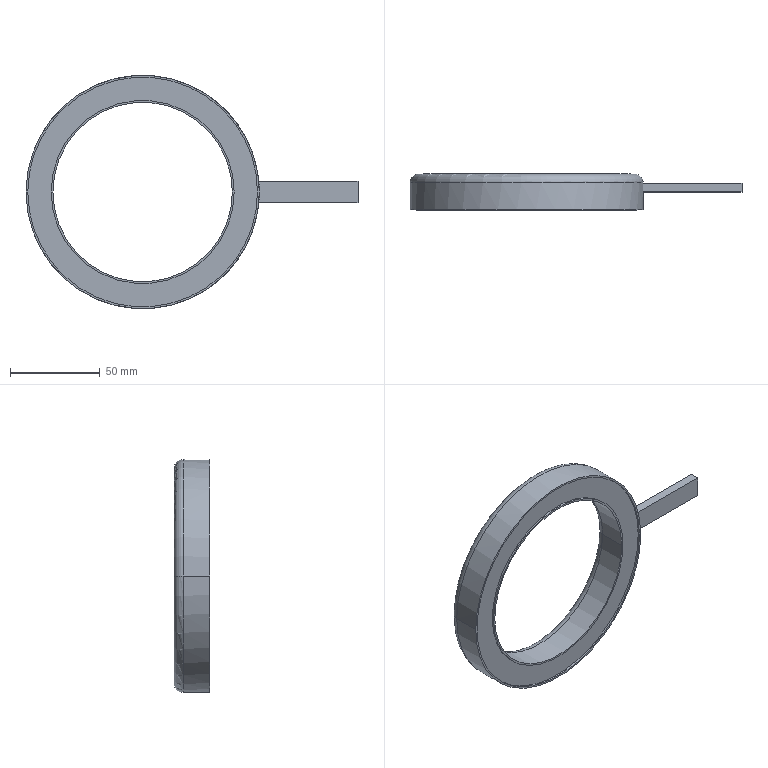Component | SolidWorks | FillLight-1 | 1 solid | 21 faces | box 185 x 20 x 130 mm | volume 103117 mm3 | plane 9 | cylinder 8 | torus 4 | commonest cylinder face diameters 102 x2 128 x2 100 x2 130 x2
STEP:
#1=CARTESIAN_POINT('',(8.917,22.343,-0.));
#2=VERTEX_POINT('',#1);
#3=CARTESIAN_POINT('',(4.902,22.343,-0.));
#4=VERTEX_POINT('',#3);
#5=CARTESIAN_POINT('',(6.909,22.343,-0.));
#6=DIRECTION('',(-0.,-1.,0.));
#7=DIRECTION('',(1.,0.,0.));
#8=AXIS2_PLACEMENT_3D('',#5,#6,#7);
#9=CIRCLE('',#8,2.008);
#10=EDGE_CURVE('',#2,#4,#9,.T.);
#11=ORIENTED_EDGE('',*,*,#10,.T.);
#12=CARTESIAN_POINT('',(4.902,22.303,-0.));
#13=VERTEX_POINT('',#12);
#14=CARTESIAN_POINT('',(4.902,22.343,-0.));
#15=DIRECTION('',(-0.,-1.,0.));
#16=VECTOR('',#15,39.37);
#17=LINE('',#14,#16);
#18=EDGE_CURVE('',#4,#13,#17,.T.);
#19=ORIENTED_EDGE('',*,*,#18,.T.);
#20=CARTESIAN_POINT('',(8.917,22.303,-0.));
#21=VERTEX_POINT('',#20);
#22=CARTESIAN_POINT('',(6.909,22.303,-0.));
#23=DIRECTION('',(-0.,-1.,0.));
#24=DIRECTION('',(1.,0.,0.));
#25=AXIS2_PLACEMENT_3D('',#22,#23,#24);
#26=CIRCLE('',#25,2.008);
#27=EDGE_CURVE('',#21,#13,#26,.T.);
#28=ORIENTED_EDGE('',*,*,#27,.F.);
#29=CARTESIAN_POINT('',(8.917,22.343,-0.));
#30=DIRECTION('',(-0.,-1.,0.));
#31=VECTOR('',#30,39.37);
#32=LINE('',#29,#31);
#33=EDGE_CURVE('',#2,#21,#32,.T.);
#34=ORIENTED_EDGE('',*,*,#33,.F.);
#35=EDGE_LOOP('',(#11,#19,#28,#34));
#36=FACE_OUTER_BOUND('',#35,.T.);
#37=CARTESIAN_POINT('',(6.909,22.343,-0.));
#38=DIRECTION('',(-0.,-1.,0.));
#39=DIRECTION('',(1.,0.,0.));
#40=AXIS2_PLACEMENT_3D('',#37,#38,#39);
#41=CYLINDRICAL_SURFACE('',#40,2.008);
#42=ADVANCED_FACE('',(#36),#41,.T.);
#43=CARTESIAN_POINT('',(4.39,22.343,-0.));
#44=VERTEX_POINT('',#43);
#45=CARTESIAN_POINT('',(9.429,22.343,-0.));
#46=VERTEX_POINT('',#45);
#47=CARTESIAN_POINT('',(6.909,22.343,-0.));
#48=DIRECTION('',(-0.,-1.,0.));
#49=DIRECTION('',(1.,0.,0.));
#50=AXIS2_PLACEMENT_3D('',#47,#48,#49);
#51=CIRCLE('',#50,2.52);
#52=EDGE_CURVE('',#44,#46,#51,.T.);
#53=ORIENTED_EDGE('',*,*,#52,.F.);
#54=CARTESIAN_POINT('',(4.39,22.303,-0.));
#55=VERTEX_POINT('',#54);
#56=CARTESIAN_POINT('',(4.39,22.343,-0.));
#57=DIRECTION('',(-0.,-1.,0.));
#58=VECTOR('',#57,39.37);
#59=LINE('',#56,#58);
#60=EDGE_CURVE('',#44,#55,#59,.T.);
#61=ORIENTED_EDGE('',*,*,#60,.T.);
#62=CARTESIAN_POINT('',(9.429,22.303,-0.));
#63=VERTEX_POINT('',#62);
#64=CARTESIAN_POINT('',(6.909,22.303,-0.));
#65=DIRECTION('',(-0.,-1.,0.));
#66=DIRECTION('',(1.,0.,0.));
#67=AXIS2_PLACEMENT_3D('',#64,#65,#66);
#68=CIRCLE('',#67,2.52);
#69=EDGE_CURVE('',#55,#63,#68,.T.);
#70=ORIENTED_EDGE('',*,*,#69,.T.);
#71=CARTESIAN_POINT('',(9.429,22.343,-0.));
#72=DIRECTION('',(-0.,-1.,0.));
#73=VECTOR('',#72,39.37);
#74=LINE('',#71,#73);
#75=EDGE_CURVE('',#46,#63,#74,.T.);
#76=ORIENTED_EDGE('',*,*,#75,.F.);
#77=EDGE_LOOP('',(#53,#61,#70,#76));
#78=FACE_OUTER_BOUND('',#77,.T.);
#79=CARTESIAN_POINT('',(6.909,22.343,-0.));
#80=DIRECTION('',(-0.,-1.,0.));
#81=DIRECTION('',(1.,0.,0.));
#82=AXIS2_PLACEMENT_3D('',#79,#80,#81);
#83=CYLINDRICAL_SURFACE('',#82,2.52);
#84=ADVANCED_FACE('',(#78),#83,.F.);
#85=CARTESIAN_POINT('',(9.075,23.091,-0.));
#86=VERTEX_POINT('',#85);
#87=CARTESIAN_POINT('',(4.744,23.091,-0.));
#88=VERTEX_POINT('',#87);
#89=CARTESIAN_POINT('',(6.909,23.091,-0.));
#90=DIRECTION('',(-0.,-1.,0.));
#91=DIRECTION('',(-1.,0.,0.));
#92=AXIS2_PLACEMENT_3D('',#89,#90,#91);
#93=CIRCLE('',#92,2.165);
#94=EDGE_CURVE('',#86,#88,#93,.T.);
#95=ORIENTED_EDGE('',*,*,#94,.F.);
#96=CARTESIAN_POINT('',(8.878,22.894,-0.));
#97=VERTEX_POINT('',#96);
#98=CARTESIAN_POINT('',(9.075,22.894,-0.));
#99=DIRECTION('',(-0.,0.,1.));
#100=DIRECTION('',(1.,0.,0.));
#101=AXIS2_PLACEMENT_3D('',#98,#99,#100);
#102=CIRCLE('',#101,0.1969);
#103=EDGE_CURVE('',#86,#97,#102,.T.);
#104=ORIENTED_EDGE('',*,*,#103,.T.);
#105=CARTESIAN_POINT('',(4.941,22.894,-0.));
#106=VERTEX_POINT('',#105);
#107=CARTESIAN_POINT('',(6.909,22.894,-0.));
#108=DIRECTION('',(0.,1.,0.));
#109=DIRECTION('',(-1.,0.,0.));
#110=AXIS2_PLACEMENT_3D('',#107,#108,#109);
#111=CIRCLE('',#110,1.969);
#112=EDGE_CURVE('',#106,#97,#111,.T.);
#113=ORIENTED_EDGE('',*,*,#112,.F.);
#114=CARTESIAN_POINT('',(4.744,22.894,-0.));
#115=DIRECTION('',(0.,-0.,-1.));
#116=DIRECTION('',(-1.,0.,0.));
#117=AXIS2_PLACEMENT_3D('',#114,#115,#116);
#118=CIRCLE('',#117,0.1969);
#119=EDGE_CURVE('',#88,#106,#118,.T.);
#120=ORIENTED_EDGE('',*,*,#119,.F.);
#121=EDGE_LOOP('',(#95,#104,#113,#120));
#122=FACE_OUTER_BOUND('',#121,.T.);
#123=CARTESIAN_POINT('',(6.909,22.894,-0.));
#124=DIRECTION('',(0.,1.,0.));
#125=DIRECTION('',(-1.,0.,0.));
#126=AXIS2_PLACEMENT_3D('',#123,#124,#125);
#127=TOROIDAL_SURFACE('',#126,2.165,0.1969);
#128=ADVANCED_FACE('',(#122),#127,.T.);
#129=CARTESIAN_POINT('',(9.458,22.894,0.2362));
#130=VERTEX_POINT('',#129);
#131=CARTESIAN_POINT('',(9.469,22.894,-0.));
#132=VERTEX_POINT('',#131);
#133=CARTESIAN_POINT('',(6.909,22.894,-0.));
#134=DIRECTION('',(0.,1.,0.));
#135=DIRECTION('',(-1.,0.,0.));
#136=AXIS2_PLACEMENT_3D('',#133,#134,#135);
#137=CIRCLE('',#136,2.559);
#138=EDGE_CURVE('',#130,#132,#137,.T.);
#139=ORIENTED_EDGE('',*,*,#138,.T.);
#140=CARTESIAN_POINT('',(9.272,23.091,-0.));
#141=VERTEX_POINT('',#140);
#142=CARTESIAN_POINT('',(9.272,22.894,-0.));
#143=DIRECTION('',(-0.,0.,1.));
#144=DIRECTION('',(1.,0.,0.));
#145=AXIS2_PLACEMENT_3D('',#142,#143,#144);
#146=CIRCLE('',#145,0.1969);
#147=EDGE_CURVE('',#132,#141,#146,.T.);
#148=ORIENTED_EDGE('',*,*,#147,.T.);
#149=CARTESIAN_POINT('',(4.547,23.091,-0.));
#150=VERTEX_POINT('',#149);
#151=CARTESIAN_POINT('',(6.909,23.091,-0.));
#152=DIRECTION('',(0.,1.,0.));
#153=DIRECTION('',(-1.,0.,0.));
#154=AXIS2_PLACEMENT_3D('',#151,#152,#153);
#155=CIRCLE('',#154,2.362);
#156=EDGE_CURVE('',#150,#141,#155,.T.);
#157=ORIENTED_EDGE('',*,*,#156,.F.);
#158=CARTESIAN_POINT('',(4.35,22.894,-0.));
#159=VERTEX_POINT('',#158);
#160=CARTESIAN_POINT('',(4.547,22.894,-0.));
#161=DIRECTION('',(0.,-0.,-1.));
#162=DIRECTION('',(-1.,0.,0.));
#163=AXIS2_PLACEMENT_3D('',#160,#161,#162);
#164=CIRCLE('',#163,0.1969);
#165=EDGE_CURVE('',#159,#150,#164,.T.);
#166=ORIENTED_EDGE('',*,*,#165,.F.);
#167=CARTESIAN_POINT('',(6.909,22.894,-0.));
#168=DIRECTION('',(-0.,-1.,0.));
#169=DIRECTION('',(-1.,0.,0.));
#170=AXIS2_PLACEMENT_3D('',#167,#168,#169);
#171=CIRCLE('',#170,2.559);
#172=EDGE_CURVE('',#130,#159,#171,.T.);
#173=ORIENTED_EDGE('',*,*,#172,.F.);
#174=EDGE_LOOP('',(#139,#148,#157,#166,#173));
#175=FACE_OUTER_BOUND('',#174,.T.);
#176=CARTESIAN_POINT('',(6.909,22.894,-0.));
#177=DIRECTION('',(0.,1.,0.));
#178=DIRECTION('',(-1.,0.,0.));
#179=AXIS2_PLACEMENT_3D('',#176,#177,#178);
#180=TOROIDAL_SURFACE('',#179,2.362,0.1969);
#181=ADVANCED_FACE('',(#175),#180,.T.);
#182=CARTESIAN_POINT('',(8.878,22.303,-0.));
#183=VERTEX_POINT('',#182);
#184=CARTESIAN_POINT('',(4.941,22.303,-0.));
#185=VERTEX_POINT('',#184);
#186=CARTESIAN_POINT('',(6.909,22.303,-0.));
#187=DIRECTION('',(0.,1.,0.));
#188=DIRECTION('',(-1.,0.,0.));
#189=AXIS2_PLACEMENT_3D('',#186,#187,#188);
#190=CIRCLE('',#189,1.969);
#191=EDGE_CURVE('',#183,#185,#190,.T.);
#192=ORIENTED_EDGE('',*,*,#191,.F.);
#193=CARTESIAN_POINT('',(8.878,22.303,-0.));
#194=DIRECTION('',(0.,1.,0.));
#195=VECTOR('',#194,39.37);
#196=LINE('',#193,#195);
#197=EDGE_CURVE('',#183,#97,#196,.T.);
#198=ORIENTED_EDGE('',*,*,#197,.T.);
#199=CARTESIAN_POINT('',(6.909,22.894,-0.));
#200=DIRECTION('',(0.,1.,0.));
#201=DIRECTION('',(-1.,0.,0.));
#202=AXIS2_PLACEMENT_3D('',#199,#200,#201);
#203=CIRCLE('',#202,1.969);
#204=EDGE_CURVE('',#97,#106,#203,.T.);
#205=ORIENTED_EDGE('',*,*,#204,.T.);
#206=CARTESIAN_POINT('',(4.941,22.303,-0.));
#207=DIRECTION('',(0.,1.,0.));
#208=VECTOR('',#207,39.37);
#209=LINE('',#206,#208);
#210=EDGE_CURVE('',#185,#106,#209,.T.);
#211=ORIENTED_EDGE('',*,*,#210,.F.);
#212=EDGE_LOOP('',(#192,#198,#205,#211));
#213=FACE_OUTER_BOUND('',#212,.T.);
#214=CARTESIAN_POINT('',(6.909,22.303,-0.));
#215=DIRECTION('',(0.,1.,0.));
#216=DIRECTION('',(-1.,0.,0.));
#217=AXIS2_PLACEMENT_3D('',#214,#215,#216);
#218=CYLINDRICAL_SURFACE('',#217,1.969);
#219=ADVANCED_FACE('',(#213),#218,.F.);
#220=CARTESIAN_POINT('',(4.35,22.303,-0.));
#221=VERTEX_POINT('',#220);
#222=CARTESIAN_POINT('',(9.469,22.303,-0.));
#223=VERTEX_POINT('',#222);
#224=CARTESIAN_POINT('',(6.909,22.303,-0.));
#225=DIRECTION('',(0.,1.,0.));
#226=DIRECTION('',(-1.,0.,0.));
#227=AXIS2_PLACEMENT_3D('',#224,#225,#226);
#228=CIRCLE('',#227,2.559);
#229=EDGE_CURVE('',#221,#223,#228,.T.);
#230=ORIENTED_EDGE('',*,*,#229,.T.);
#231=CARTESIAN_POINT('',(9.469,22.697,-0.));
#232=VERTEX_POINT('',#231);
#233=CARTESIAN_POINT('',(9.469,22.303,-0.));
#234=DIRECTION('',(0.,1.,0.));
#235=VECTOR('',#234,39.37);
#236=LINE('',#233,#235);
#237=EDGE_CURVE('',#223,#232,#236,.T.);
#238=ORIENTED_EDGE('',*,*,#237,.T.);
#239=CARTESIAN_POINT('',(9.458,22.697,0.2362));
#240=VERTEX_POINT('',#239);
#241=CARTESIAN_POINT('',(6.909,22.697,-0.));
#242=DIRECTION('',(0.,1.,0.));
#243=DIRECTION('',(-1.,0.,0.));
#244=AXIS2_PLACEMENT_3D('',#241,#242,#243);
#245=CIRCLE('',#244,2.559);
#246=EDGE_CURVE('',#240,#232,#245,.T.);
#247=ORIENTED_EDGE('',*,*,#246,.F.);
#248=CARTESIAN_POINT('',(9.458,22.303,0.2362));
#249=DIRECTION('',(-0.,-1.,0.));
#250=VECTOR('',#249,39.37);
#251=LINE('',#248,#250);
#252=EDGE_CURVE('',#130,#240,#251,.T.);
#253=ORIENTED_EDGE('',*,*,#252,.F.);
#254=ORIENTED_EDGE('',*,*,#172,.T.);
#255=CARTESIAN_POINT('',(4.35,22.303,-0.));
#256=DIRECTION('',(0.,1.,0.));
#257=VECTOR('',#256,39.37);
#258=LINE('',#255,#257);
#259=EDGE_CURVE('',#221,#159,#258,.T.);
#260=ORIENTED_EDGE('',*,*,#259,.F.);
#261=EDGE_LOOP('',(#230,#238,#247,#253,#254,#260));
#262=FACE_OUTER_BOUND('',#261,.T.);
#263=CARTESIAN_POINT('',(6.909,22.303,-0.));
#264=DIRECTION('',(0.,1.,0.));
#265=DIRECTION('',(-1.,0.,0.));
#266=AXIS2_PLACEMENT_3D('',#263,#264,#265);
#267=CYLINDRICAL_SURFACE('',#266,2.559);
#268=ADVANCED_FACE('',(#262),#267,.T.);
#269=CARTESIAN_POINT('',(6.909,22.303,-0.));
#270=DIRECTION('',(0.,1.,0.));
#271=DIRECTION('',(-1.,0.,0.));
#272=AXIS2_PLACEMENT_3D('',#269,#270,#271);
#273=CIRCLE('',#272,1.969);
#274=EDGE_CURVE('',#185,#183,#273,.T.);
#275=ORIENTED_EDGE('',*,*,#274,.T.);
#276=ORIENTED_EDGE('',*,*,#191,.T.);
#277=EDGE_LOOP('',(#275,#276));
#278=FACE_BOUND('',#277,.T.);
#279=ORIENTED_EDGE('',*,*,#27,.T.);
#280=CARTESIAN_POINT('',(6.909,22.303,-0.));
#281=DIRECTION('',(-0.,-1.,0.));
#282=DIRECTION('',(1.,0.,0.));
#283=AXIS2_PLACEMENT_3D('',#280,#281,#282);
#284=CIRCLE('',#283,2.008);
#285=EDGE_CURVE('',#13,#21,#284,.T.);
#286=ORIENTED_EDGE('',*,*,#285,.T.);
#287=EDGE_LOOP('',(#279,#286));
#288=FACE_OUTER_BOUND('',#287,.T.);
#289=CARTESIAN_POINT('',(6.909,22.303,-0.));
#290=DIRECTION('',(0.,1.,0.));
#291=DIRECTION('',(-1.,0.,-0.));
#292=AXIS2_PLACEMENT_3D('',#289,#290,#291);
#293=PLANE('',#292);
#294=ADVANCED_FACE('',(#278,#288),#293,.F.);
#295=ORIENTED_EDGE('',*,*,#138,.F.);
#296=CARTESIAN_POINT('',(11.634,22.894,0.2362));
#297=VERTEX_POINT('',#296);
#298=CARTESIAN_POINT('',(6.909,22.894,0.2362));
#299=DIRECTION('',(1.,-0.,0.));
#300=VECTOR('',#299,39.37);
#301=LINE('',#298,#300);
#302=EDGE_CURVE('',#130,#297,#301,.T.);
#303=ORIENTED_EDGE('',*,*,#302,.T.);
#304=CARTESIAN_POINT('',(11.634,22.894,-0.2362));
#305=VERTEX_POINT('',#304);
#306=CARTESIAN_POINT('',(11.634,22.894,-0.2362));
#307=DIRECTION('',(0.,0.,-1.));
#308=VECTOR('',#307,39.37);
#309=LINE('',#306,#308);
#310=EDGE_CURVE('',#297,#305,#309,.T.);
#311=ORIENTED_EDGE('',*,*,#310,.T.);
#312=CARTESIAN_POINT('',(9.458,22.894,-0.2362));
#313=VERTEX_POINT('',#312);
#314=CARTESIAN_POINT('',(6.909,22.894,-0.2362));
#315=DIRECTION('',(1.,-0.,0.));
#316=VECTOR('',#315,39.37);
#317=LINE('',#314,#316);
#318=EDGE_CURVE('',#313,#305,#317,.T.);
#319=ORIENTED_EDGE('',*,*,#318,.F.);
#320=CARTESIAN_POINT('',(6.909,22.894,-0.));
#321=DIRECTION('',(0.,1.,0.));
#322=DIRECTION('',(-1.,0.,0.));
#323=AXIS2_PLACEMENT_3D('',#320,#321,#322);
#324=CIRCLE('',#323,2.559);
#325=EDGE_CURVE('',#132,#313,#324,.T.);
#326=ORIENTED_EDGE('',*,*,#325,.F.);
#327=EDGE_LOOP('',(#295,#303,#311,#319,#326));
#328=FACE_OUTER_BOUND('',#327,.T.);
#329=CARTESIAN_POINT('',(6.909,22.894,-0.2362));
#330=DIRECTION('',(-0.,-1.,-0.));
#331=DIRECTION('',(1.,-0.,0.));
#332=AXIS2_PLACEMENT_3D('',#329,#330,#331);
#333=PLANE('',#332);
#334=ADVANCED_FACE('',(#328),#333,.F.);
#335=ORIENTED_EDGE('',*,*,#302,.F.);
#336=ORIENTED_EDGE('',*,*,#252,.T.);
#337=CARTESIAN_POINT('',(11.634,22.697,0.2362));
#338=VERTEX_POINT('',#337);
#339=CARTESIAN_POINT('',(6.909,22.697,0.2362));
#340=DIRECTION('',(1.,-0.,0.));
#341=VECTOR('',#340,39.37);
#342=LINE('',#339,#341);
#343=EDGE_CURVE('',#240,#338,#342,.T.);
#344=ORIENTED_EDGE('',*,*,#343,.T.);
#345=CARTESIAN_POINT('',(11.634,22.894,0.2362));
#346=DIRECTION('',(0.,1.,0.));
#347=VECTOR('',#346,39.37);
#348=LINE('',#345,#347);
#349=EDGE_CURVE('',#338,#297,#348,.T.);
#350=ORIENTED_EDGE('',*,*,#349,.T.);
#351=EDGE_LOOP('',(#335,#336,#344,#350));
#352=FACE_OUTER_BOUND('',#351,.T.);
#353=CARTESIAN_POINT('',(6.909,22.894,0.2362));
#354=DIRECTION('',(0.,-0.,-1.));
#355=DIRECTION('',(-1.,0.,-0.));
#356=AXIS2_PLACEMENT_3D('',#353,#354,#355);
#357=PLANE('',#356);
#358=ADVANCED_FACE('',(#352),#357,.F.);
#359=CARTESIAN_POINT('',(9.458,22.697,-0.2362));
#360=VERTEX_POINT('',#359);
#361=CARTESIAN_POINT('',(11.634,22.697,-0.2362));
#362=VERTEX_POINT('',#361);
#363=CARTESIAN_POINT('',(6.909,22.697,-0.2362));
#364=DIRECTION('',(1.,-0.,0.));
#365=VECTOR('',#364,39.37);
#366=LINE('',#363,#365);
#367=EDGE_CURVE('',#360,#362,#366,.T.);
#368=ORIENTED_EDGE('',*,*,#367,.F.);
#369=CARTESIAN_POINT('',(9.458,22.303,-0.2362));
#370=DIRECTION('',(0.,1.,0.));
#371=VECTOR('',#370,39.37);
#372=LINE('',#369,#371);
#373=EDGE_CURVE('',#360,#313,#372,.T.);
#374=ORIENTED_EDGE('',*,*,#373,.T.);
#375=ORIENTED_EDGE('',*,*,#318,.T.);
#376=CARTESIAN_POINT('',(11.634,22.894,-0.2362));
#377=DIRECTION('',(-0.,-1.,0.));
#378=VECTOR('',#377,39.37);
#379=LINE('',#376,#378);
#380=EDGE_CURVE('',#305,#362,#379,.T.);
#381=ORIENTED_EDGE('',*,*,#380,.T.);
#382=EDGE_LOOP('',(#368,#374,#375,#381));
#383=FACE_OUTER_BOUND('',#382,.T.);
#384=CARTESIAN_POINT('',(6.909,22.894,-0.2362));
#385=DIRECTION('',(-0.,0.,1.));
#386=DIRECTION('',(1.,-0.,0.));
#387=AXIS2_PLACEMENT_3D('',#384,#385,#386);
#388=PLANE('',#387);
#389=ADVANCED_FACE('',(#383),#388,.F.);
#390=ORIENTED_EDGE('',*,*,#343,.F.);
#391=ORIENTED_EDGE('',*,*,#246,.T.);
#392=CARTESIAN_POINT('',(6.909,22.697,-0.));
#393=DIRECTION('',(0.,1.,0.));
#394=DIRECTION('',(-1.,0.,0.));
#395=AXIS2_PLACEMENT_3D('',#392,#393,#394);
#396=CIRCLE('',#395,2.559);
#397=EDGE_CURVE('',#232,#360,#396,.T.);
#398=ORIENTED_EDGE('',*,*,#397,.T.);
#399=ORIENTED_EDGE('',*,*,#367,.T.);
#400=CARTESIAN_POINT('',(11.634,22.697,-0.2362));
#401=DIRECTION('',(-0.,0.,1.));
#402=VECTOR('',#401,39.37);
#403=LINE('',#400,#402);
#404=EDGE_CURVE('',#362,#338,#403,.T.);
#405=ORIENTED_EDGE('',*,*,#404,.T.);
#406=EDGE_LOOP('',(#390,#391,#398,#399,#405));
#407=FACE_OUTER_BOUND('',#406,.T.);
#408=CARTESIAN_POINT('',(6.909,22.697,-0.2362));
#409=DIRECTION('',(0.,1.,0.));
#410=DIRECTION('',(-1.,0.,-0.));
#411=AXIS2_PLACEMENT_3D('',#408,#409,#410);
#412=PLANE('',#411);
#413=ADVANCED_FACE('',(#407),#412,.F.);
#414=ORIENTED_EDGE('',*,*,#349,.F.);
#415=ORIENTED_EDGE('',*,*,#404,.F.);
#416=ORIENTED_EDGE('',*,*,#380,.F.);
#417=ORIENTED_EDGE('',*,*,#310,.F.);
#418=EDGE_LOOP('',(#414,#415,#416,#417));
#419=FACE_OUTER_BOUND('',#418,.T.);
#420=CARTESIAN_POINT('',(11.634,22.795,-0.));
#421=DIRECTION('',(-1.,0.,-0.));
#422=DIRECTION('',(-0.,0.,1.));
#423=AXIS2_PLACEMENT_3D('',#420,#421,#422);
#424=PLANE('',#423);
#425=ADVANCED_FACE('',(#419),#424,.F.);
#426=ORIENTED_EDGE('',*,*,#237,.F.);
#427=CARTESIAN_POINT('',(6.909,22.303,-0.));
#428=DIRECTION('',(0.,1.,0.));
#429=DIRECTION('',(-1.,0.,0.));
#430=AXIS2_PLACEMENT_3D('',#427,#428,#429);
#431=CIRCLE('',#430,2.559);
#432=EDGE_CURVE('',#223,#221,#431,.T.);
#433=ORIENTED_EDGE('',*,*,#432,.T.);
#434=ORIENTED_EDGE('',*,*,#259,.T.);
#435=CARTESIAN_POINT('',(6.909,22.894,-0.));
#436=DIRECTION('',(-0.,-1.,0.));
#437=DIRECTION('',(-1.,0.,0.));
#438=AXIS2_PLACEMENT_3D('',#435,#436,#437);
#439=CIRCLE('',#438,2.559);
#440=EDGE_CURVE('',#159,#313,#439,.T.);
#441=ORIENTED_EDGE('',*,*,#440,.T.);
#442=ORIENTED_EDGE('',*,*,#373,.F.);
#443=ORIENTED_EDGE('',*,*,#397,.F.);
#444=EDGE_LOOP('',(#426,#433,#434,#441,#442,#443));
#445=FACE_OUTER_BOUND('',#444,.T.);
#446=CARTESIAN_POINT('',(6.909,22.303,-0.));
#447=DIRECTION('',(0.,1.,0.));
#448=DIRECTION('',(-1.,0.,0.));
#449=AXIS2_PLACEMENT_3D('',#446,#447,#448);
#450=CYLINDRICAL_SURFACE('',#449,2.559);
#451=ADVANCED_FACE('',(#445),#450,.T.);
#452=ORIENTED_EDGE('',*,*,#197,.F.);
#453=ORIENTED_EDGE('',*,*,#274,.F.);
#454=ORIENTED_EDGE('',*,*,#210,.T.);
#455=ORIENTED_EDGE('',*,*,#112,.T.);
#456=EDGE_LOOP('',(#452,#453,#454,#455));
#457=FACE_OUTER_BOUND('',#456,.T.);
#458=CARTESIAN_POINT('',(6.909,22.303,-0.));
#459=DIRECTION('',(0.,1.,0.));
#460=DIRECTION('',(-1.,0.,0.));
#461=AXIS2_PLACEMENT_3D('',#458,#459,#460);
#462=CYLINDRICAL_SURFACE('',#461,1.969);
#463=ADVANCED_FACE('',(#457),#462,.F.);
#464=CARTESIAN_POINT('',(6.909,22.303,-0.));
#465=DIRECTION('',(-0.,-1.,0.));
#466=DIRECTION('',(1.,0.,0.));
#467=AXIS2_PLACEMENT_3D('',#464,#465,#466);
#468=CIRCLE('',#467,2.52);
#469=EDGE_CURVE('',#63,#55,#468,.T.);
#470=ORIENTED_EDGE('',*,*,#469,.F.);
#471=ORIENTED_EDGE('',*,*,#69,.F.);
#472=EDGE_LOOP('',(#470,#471));
#473=FACE_BOUND('',#472,.T.);
#474=ORIENTED_EDGE('',*,*,#229,.F.);
#475=ORIENTED_EDGE('',*,*,#432,.F.);
#476=EDGE_LOOP('',(#474,#475));
#477=FACE_OUTER_BOUND('',#476,.T.);
#478=CARTESIAN_POINT('',(6.909,22.303,-0.));
#479=DIRECTION('',(0.,1.,0.));
#480=DIRECTION('',(-1.,0.,-0.));
#481=AXIS2_PLACEMENT_3D('',#478,#479,#480);
#482=PLANE('',#481);
#483=ADVANCED_FACE('',(#473,#477),#482,.F.);
#484=ORIENTED_EDGE('',*,*,#156,.T.);
#485=CARTESIAN_POINT('',(6.909,23.091,-0.));
#486=DIRECTION('',(0.,1.,0.));
#487=DIRECTION('',(-1.,0.,0.));
#488=AXIS2_PLACEMENT_3D('',#485,#486,#487);
#489=CIRCLE('',#488,2.362);
#490=EDGE_CURVE('',#141,#150,#489,.T.);
#491=ORIENTED_EDGE('',*,*,#490,.T.);
#492=EDGE_LOOP('',(#484,#491));
#493=FACE_OUTER_BOUND('',#492,.T.);
#494=CARTESIAN_POINT('',(6.909,23.091,-0.));
#495=DIRECTION('',(-0.,-1.,0.));
#496=DIRECTION('',(-1.,0.,0.));
#497=AXIS2_PLACEMENT_3D('',#494,#495,#496);
#498=CIRCLE('',#497,2.165);
#499=EDGE_CURVE('',#88,#86,#498,.T.);
#500=ORIENTED_EDGE('',*,*,#499,.T.);
#501=ORIENTED_EDGE('',*,*,#94,.T.);
#502=EDGE_LOOP('',(#500,#501));
#503=FACE_BOUND('',#502,.T.);
#504=CARTESIAN_POINT('',(6.909,23.091,-0.));
#505=DIRECTION('',(0.,1.,0.));
#506=DIRECTION('',(-1.,0.,-0.));
#507=AXIS2_PLACEMENT_3D('',#504,#505,#506);
#508=PLANE('',#507);
#509=ADVANCED_FACE('',(#493,#503),#508,.T.);
#510=ORIENTED_EDGE('',*,*,#147,.F.);
#511=ORIENTED_EDGE('',*,*,#325,.T.);
#512=ORIENTED_EDGE('',*,*,#440,.F.);
#513=ORIENTED_EDGE('',*,*,#165,.T.);
#514=ORIENTED_EDGE('',*,*,#490,.F.);
#515=EDGE_LOOP('',(#510,#511,#512,#513,#514));
#516=FACE_OUTER_BOUND('',#515,.T.);
#517=CARTESIAN_POINT('',(6.909,22.894,-0.));
#518=DIRECTION('',(0.,1.,0.));
#519=DIRECTION('',(-1.,0.,0.));
#520=AXIS2_PLACEMENT_3D('',#517,#518,#519);
#521=TOROIDAL_SURFACE('',#520,2.362,0.1969);
#522=ADVANCED_FACE('',(#516),#521,.T.);
#523=ORIENTED_EDGE('',*,*,#103,.F.);
#524=ORIENTED_EDGE('',*,*,#499,.F.);
#525=ORIENTED_EDGE('',*,*,#119,.T.);
#526=ORIENTED_EDGE('',*,*,#204,.F.);
#527=EDGE_LOOP('',(#523,#524,#525,#526));
#528=FACE_OUTER_BOUND('',#527,.T.);
#529=CARTESIAN_POINT('',(6.909,22.894,-0.));
#530=DIRECTION('',(0.,1.,0.));
#531=DIRECTION('',(-1.,0.,0.));
#532=AXIS2_PLACEMENT_3D('',#529,#530,#531);
#533=TOROIDAL_SURFACE('',#532,2.165,0.1969);
#534=ADVANCED_FACE('',(#528),#533,.T.);
#535=ORIENTED_EDGE('',*,*,#60,.F.);
#536=CARTESIAN_POINT('',(6.909,22.343,-0.));
#537=DIRECTION('',(-0.,-1.,0.));
#538=DIRECTION('',(1.,0.,0.));
#539=AXIS2_PLACEMENT_3D('',#536,#537,#538);
#540=CIRCLE('',#539,2.52);
#541=EDGE_CURVE('',#46,#44,#540,.T.);
#542=ORIENTED_EDGE('',*,*,#541,.F.);
#543=ORIENTED_EDGE('',*,*,#75,.T.);
#544=ORIENTED_EDGE('',*,*,#469,.T.);
#545=EDGE_LOOP('',(#535,#542,#543,#544));
#546=FACE_OUTER_BOUND('',#545,.T.);
#547=CARTESIAN_POINT('',(6.909,22.343,-0.));
#548=DIRECTION('',(-0.,-1.,0.));
#549=DIRECTION('',(1.,0.,0.));
#550=AXIS2_PLACEMENT_3D('',#547,#548,#549);
#551=CYLINDRICAL_SURFACE('',#550,2.52);
#552=ADVANCED_FACE('',(#546),#551,.F.);
#553=ORIENTED_EDGE('',*,*,#10,.F.);
#554=CARTESIAN_POINT('',(6.909,22.343,-0.));
#555=DIRECTION('',(-0.,-1.,0.));
#556=DIRECTION('',(1.,0.,0.));
#557=AXIS2_PLACEMENT_3D('',#554,#555,#556);
#558=CIRCLE('',#557,2.008);
#559=EDGE_CURVE('',#4,#2,#558,.T.);
#560=ORIENTED_EDGE('',*,*,#559,.F.);
#561=EDGE_LOOP('',(#553,#560));
#562=FACE_BOUND('',#561,.T.);
#563=ORIENTED_EDGE('',*,*,#541,.T.);
#564=ORIENTED_EDGE('',*,*,#52,.T.);
#565=EDGE_LOOP('',(#563,#564));
#566=FACE_OUTER_BOUND('',#565,.T.);
#567=CARTESIAN_POINT('',(6.909,22.343,-0.));
#568=DIRECTION('',(-0.,-1.,-0.));
#569=DIRECTION('',(1.,-0.,0.));
#570=AXIS2_PLACEMENT_3D('',#567,#568,#569);
#571=PLANE('',#570);
#572=ADVANCED_FACE('',(#562,#566),#571,.T.);
#573=ORIENTED_EDGE('',*,*,#18,.F.);
#574=ORIENTED_EDGE('',*,*,#559,.T.);
#575=ORIENTED_EDGE('',*,*,#33,.T.);
#576=ORIENTED_EDGE('',*,*,#285,.F.);
#577=EDGE_LOOP('',(#573,#574,#575,#576));
#578=FACE_OUTER_BOUND('',#577,.T.);
#579=CARTESIAN_POINT('',(6.909,22.343,-0.));
#580=DIRECTION('',(-0.,-1.,0.));
#581=DIRECTION('',(1.,0.,0.));
#582=AXIS2_PLACEMENT_3D('',#579,#580,#581);
#583=CYLINDRICAL_SURFACE('',#582,2.008);
#584=ADVANCED_FACE('',(#578),#583,.T.);
#585=CLOSED_SHELL('',(#42,#84,#128,#181,#219,#268,#294,#334,#358,#389,#413,#425,#451,#463,#483,#509,#522,#534,#552,#572,#584));
#586=MANIFOLD_SOLID_BREP('',#585);
#587=CARTESIAN_POINT('',(0.,0.,0.));
#588=DIRECTION('',(0.,0.,1.));
#589=DIRECTION('',(1.,0.,0.));
#590=AXIS2_PLACEMENT_3D('',#587,#588,#589);
#591=(LENGTH_UNIT()NAMED_UNIT(*)SI_UNIT($,.METRE.));
#592=LENGTH_MEASURE_WITH_UNIT(LENGTH_MEASURE(0.0254),#591);
#593=DIMENSIONAL_EXPONENTS(1.,0.,0.,0.,0.,0.,0.);
#594=(CONVERSION_BASED_UNIT('',#592)LENGTH_UNIT()NAMED_UNIT(#593));
#595=UNCERTAINTY_MEASURE_WITH_UNIT(LENGTH_MEASURE(0.00001),#594,'','');
#596=(NAMED_UNIT(*)PLANE_ANGLE_UNIT()SI_UNIT($,.RADIAN.));
#597=(NAMED_UNIT(*)SI_UNIT($,.STERADIAN.)SOLID_ANGLE_UNIT());
#598=(GEOMETRIC_REPRESENTATION_CONTEXT(3)GLOBAL_UNCERTAINTY_ASSIGNED_CONTEXT((#595))GLOBAL_UNIT_ASSIGNED_CONTEXT((#594,#596,#597))REPRESENTATION_CONTEXT('',''));
#599=ADVANCED_BREP_SHAPE_REPRESENTATION('',(#586,#590),#598);
#600=COLOUR_RGB('',0.7922,0.8196,0.9333);
#601=FILL_AREA_STYLE_COLOUR('',#600);
#602=FILL_AREA_STYLE('',(#601));
#603=SURFACE_STYLE_FILL_AREA(#602);
#604=SURFACE_SIDE_STYLE('',(#603));
#605=SURFACE_STYLE_USAGE(.BOTH.,#604);
#606=PRESENTATION_STYLE_ASSIGNMENT((#605));
#607=STYLED_ITEM('',(#606),#586);
#608=PRESENTATION_LAYER_ASSIGNMENT('','',(#607));
#609=(LENGTH_UNIT()NAMED_UNIT(*)SI_UNIT($,.METRE.));
#610=LENGTH_MEASURE_WITH_UNIT(LENGTH_MEASURE(0.0254),#609);
#611=DIMENSIONAL_EXPONENTS(1.,0.,0.,0.,0.,0.,0.);
#612=(CONVERSION_BASED_UNIT('',#610)LENGTH_UNIT()NAMED_UNIT(#611));
#613=UNCERTAINTY_MEASURE_WITH_UNIT(LENGTH_MEASURE(0.00001),#612,'','');
#614=(NAMED_UNIT(*)PLANE_ANGLE_UNIT()SI_UNIT($,.RADIAN.));
#615=(NAMED_UNIT(*)SI_UNIT($,.STERADIAN.)SOLID_ANGLE_UNIT());
#616=(GEOMETRIC_REPRESENTATION_CONTEXT(3)GLOBAL_UNCERTAINTY_ASSIGNED_CONTEXT((#613))GLOBAL_UNIT_ASSIGNED_CONTEXT((#612,#614,#615))REPRESENTATION_CONTEXT('',''));
#617=MECHANICAL_DESIGN_GEOMETRIC_PRESENTATION_REPRESENTATION('',(#607),#616);